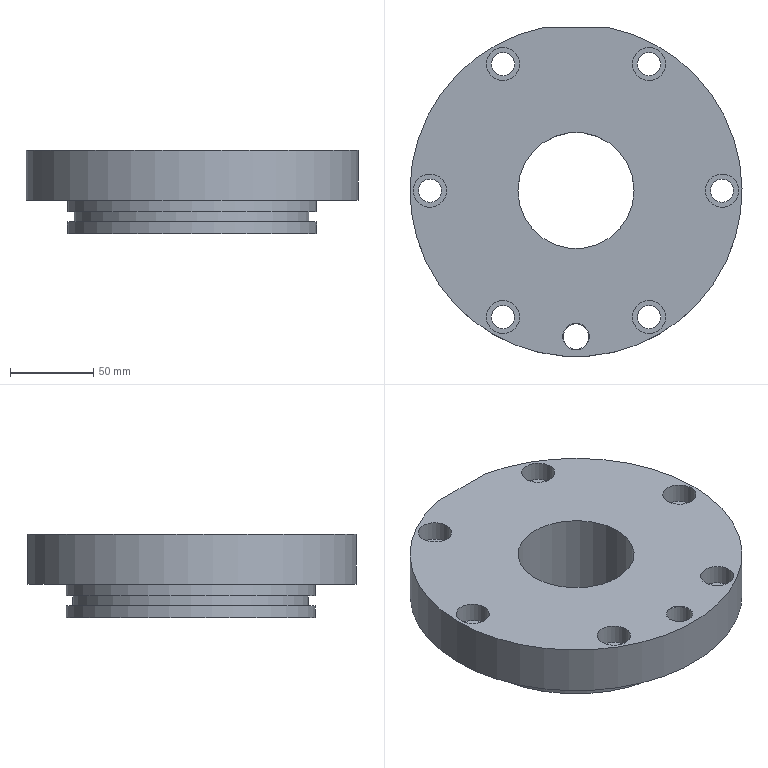Component | NX | CH3404_6-4 | 1 solid | 47 faces | volume 1013097 mm3 | cylinder 25 | plane 14 | cone 8 | commonest cylinder face diameters 14 x6 20 x6 12 x5 150 x2 200 x1 142 x1 132 x1 84 x1